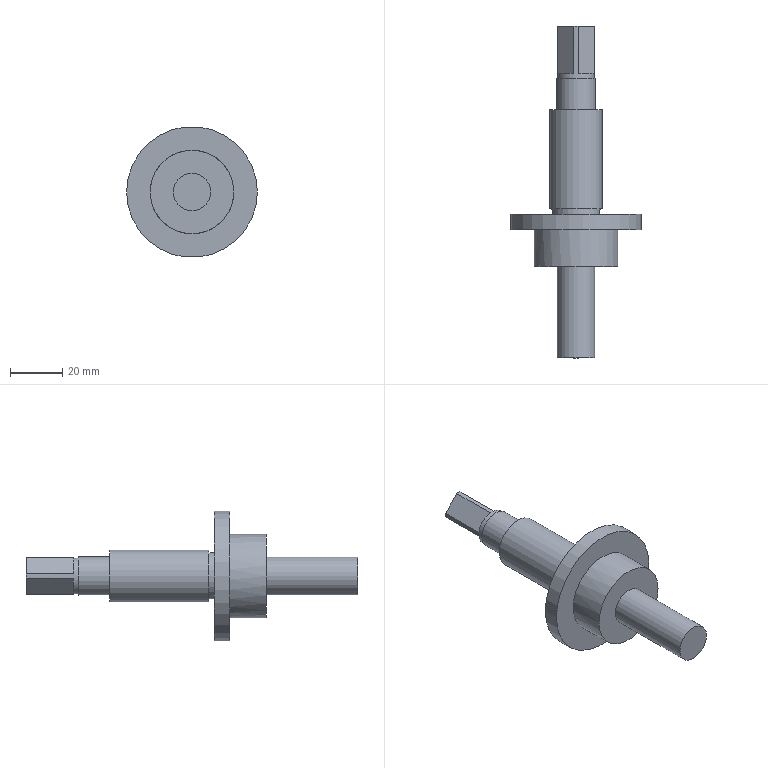Component | NX | LOCATING_MANDREL | 1 solid | 23 faces | volume 45669 mm3 | plane 16 | cylinder 7 | commonest cylinder face diameters 32 x1 50 x1 14.376 x1 18 x1 20 x1 14.782 x1 14 x1